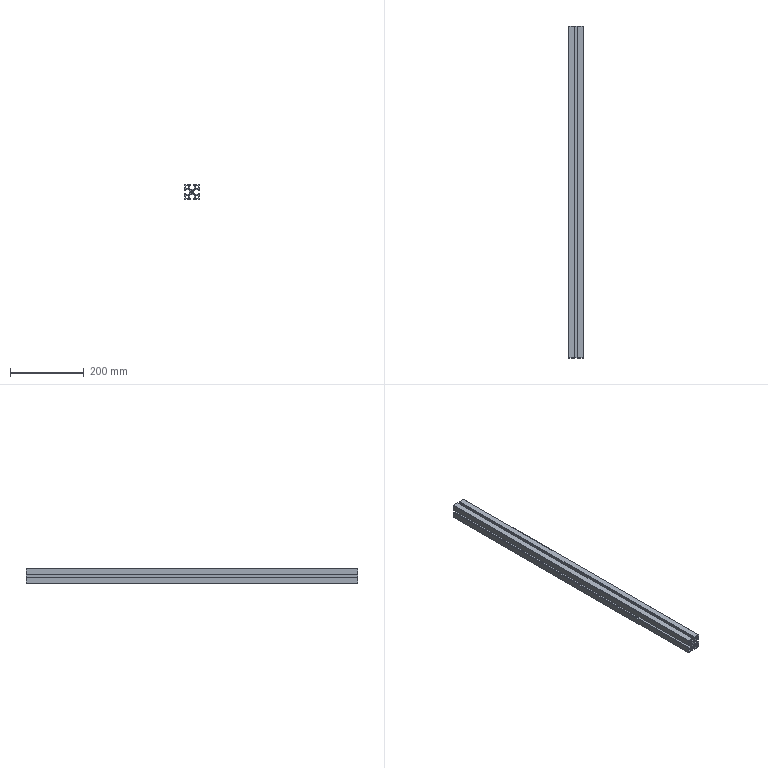Component | SolidWorks | AluminumBracket-1 | 1 solid | 56 faces | box 40 x 900 x 40 mm | volume 686166 mm3 | plane 42 | cylinder 14 | commonest cylinder face diameters 8 x8 1 x4 6.8 x2
build123d program:
from build123d import *

# Parameters (mm, degrees)
SKETCH14_R                                = 3.4
SKETCH14_R_2                              = 4
ALUMINUM_PROFILE_40_X_40GF_X_R0_5_1_DEPTH = 900


with BuildPart() as part:
    # Sketch14 → Aluminum Profile 40 X 40GF X R0.5_1 (new body)
    with BuildSketch(Plane.ZY):
        with BuildLine():
            Line((-19.5, 20), (-4, 20))
            Line((-4, 20), (-4, 17))
            Line((-4, 17), (-6, 17))
            Line((-6, 17), (-6, 7))
            Line((-6, 7), (-4, 7))
            Line((-4, 7), (-4, 4))
            Line((-4, 4), (4, 4))
            Line((4, 4), (4, 7))
            Line((4, 7), (6, 7))
            Line((6, 7), (6, 17))
            Line((6, 17), (4, 17))
            Line((4, 17), (4, 20))
            Line((4, 20), (19.5, 20))
            ThreePointArc((19.5, 20), (19.854, 19.854), (20, 19.5))
            Line((20, 19.5), (20, 4))
            Line((20, 4), (17, 4))
            Line((17, 4), (17, 6))
            Line((17, 6), (7, 6))
            Line((7, 6), (7, -6))
            Line((7, -6), (17, -6))
            Line((17, -6), (17, -4))
            Line((17, -4), (20, -4))
            Line((20, -4), (20, -19.5))
            ThreePointArc((20, -19.5), (19.854, -19.854), (19.5, -20))
            Line((19.5, -20), (4, -20))
            Line((4, -20), (4, -17))
            Line((4, -17), (6, -17))
            Line((6, -17), (6, -7))
            Line((6, -7), (-6, -7))
            Line((-6, -7), (-6, -17))
            Line((-6, -17), (-4, -17))
            Line((-4, -17), (-4, -20))
            Line((-4, -20), (-19.5, -20))
            ThreePointArc((-19.5, -20), (-19.854, -19.854), (-20, -19.5))
            Line((-20, -19.5), (-20, -4))
            Line((-20, -4), (-17, -4))
            Line((-17, -4), (-17, -6))
            Line((-17, -6), (-7, -6))
            Line((-7, -6), (-7, 6))
            Line((-7, 6), (-17, 6))
            Line((-17, 6), (-17, 4))
            Line((-17, 4), (-20, 4))
            Line((-20, 4), (-20, 19.5))
            ThreePointArc((-20, 19.5), (-19.854, 19.854), (-19.5, 20))
        make_face()
        Circle(SKETCH14_R, mode=Mode.SUBTRACT)
        with Locations((-13.435, 13.435)):
            Circle(SKETCH14_R_2, mode=Mode.SUBTRACT)
        with Locations((13.435, 13.435)):
            Circle(SKETCH14_R_2, mode=Mode.SUBTRACT)
        with Locations((13.435, -13.435)):
            Circle(SKETCH14_R_2, mode=Mode.SUBTRACT)
        with Locations((-13.435, -13.435)):
            Circle(SKETCH14_R_2, mode=Mode.SUBTRACT)
    extrude(amount=ALUMINUM_PROFILE_40_X_40GF_X_R0_5_1_DEPTH)


solid = part.part

# Placed as in the assembly
solid = solid.moved(Location((914.468, -335.334, 1356.399), (0, 0, -90)))